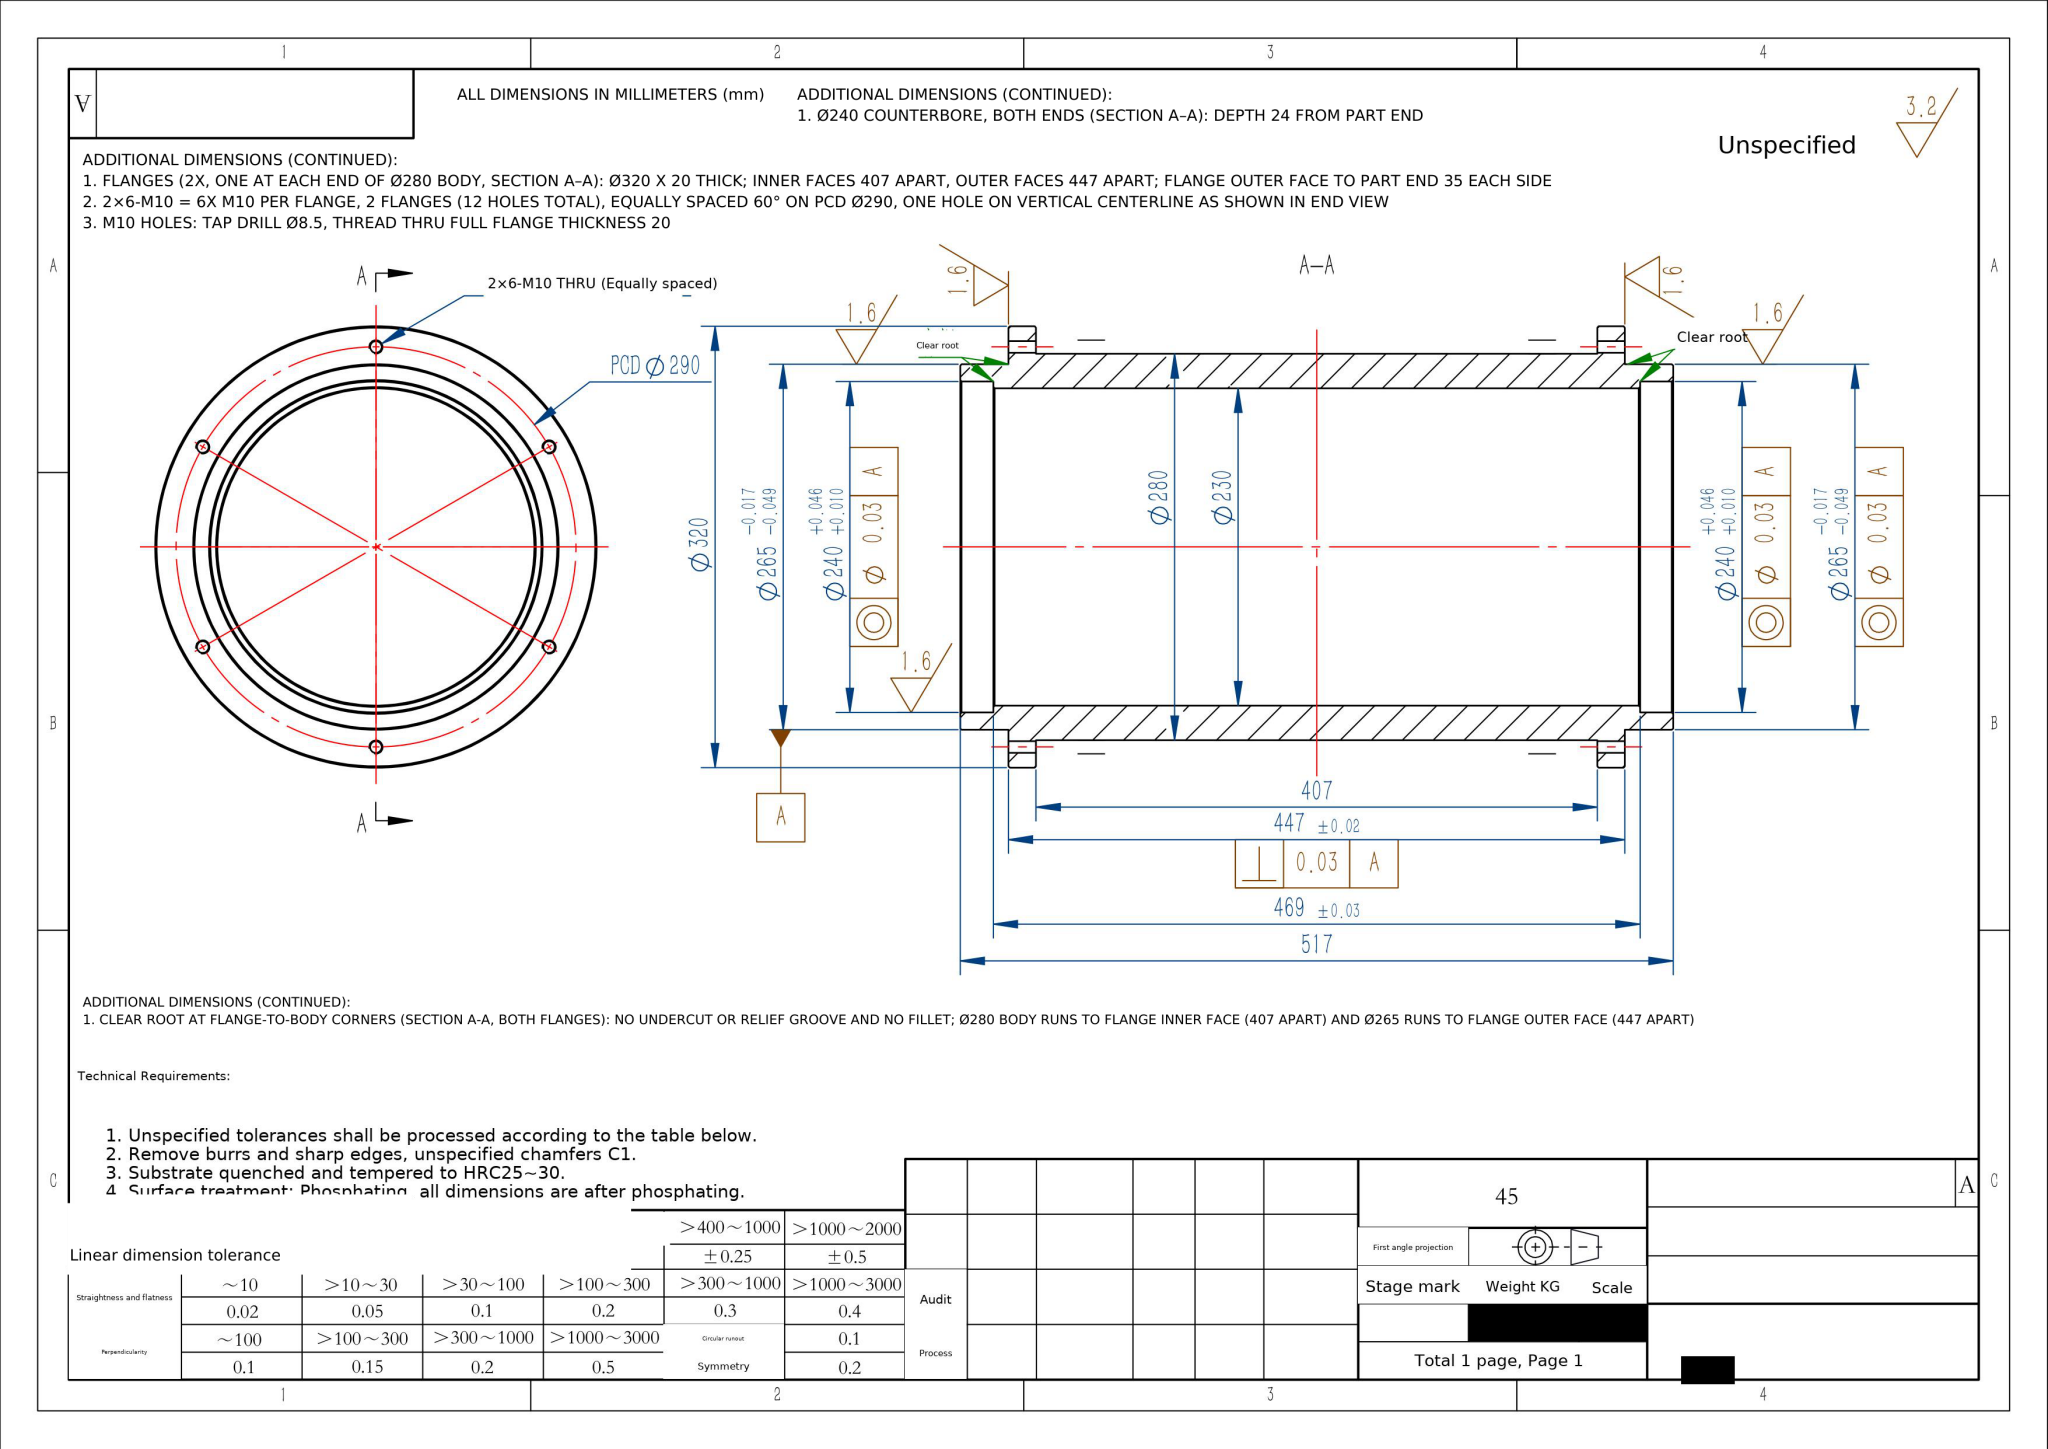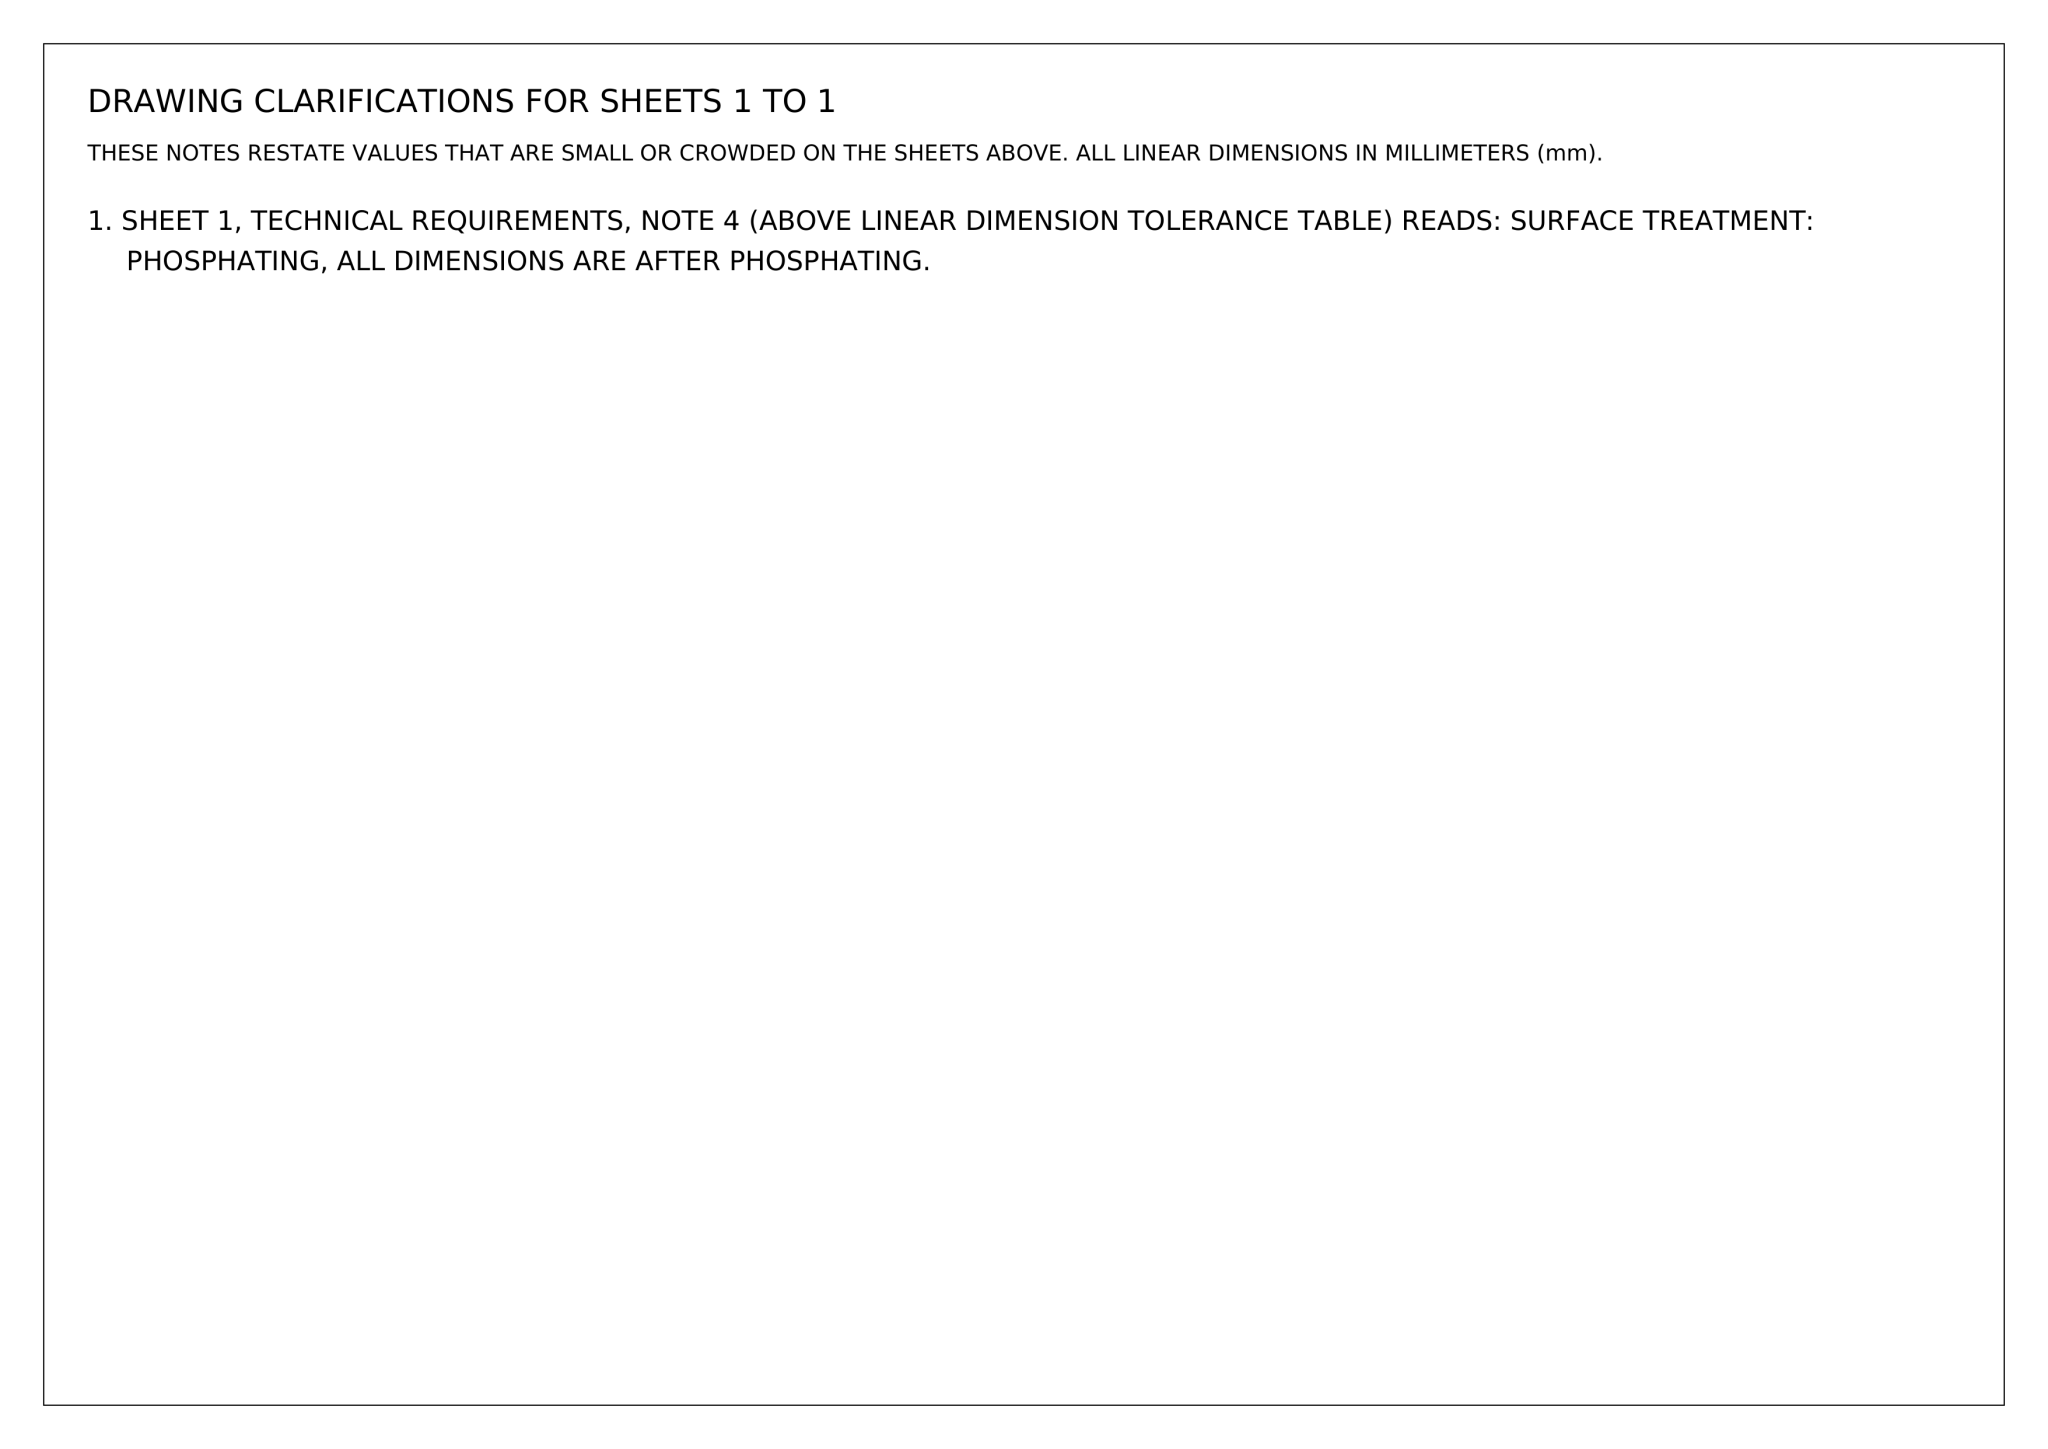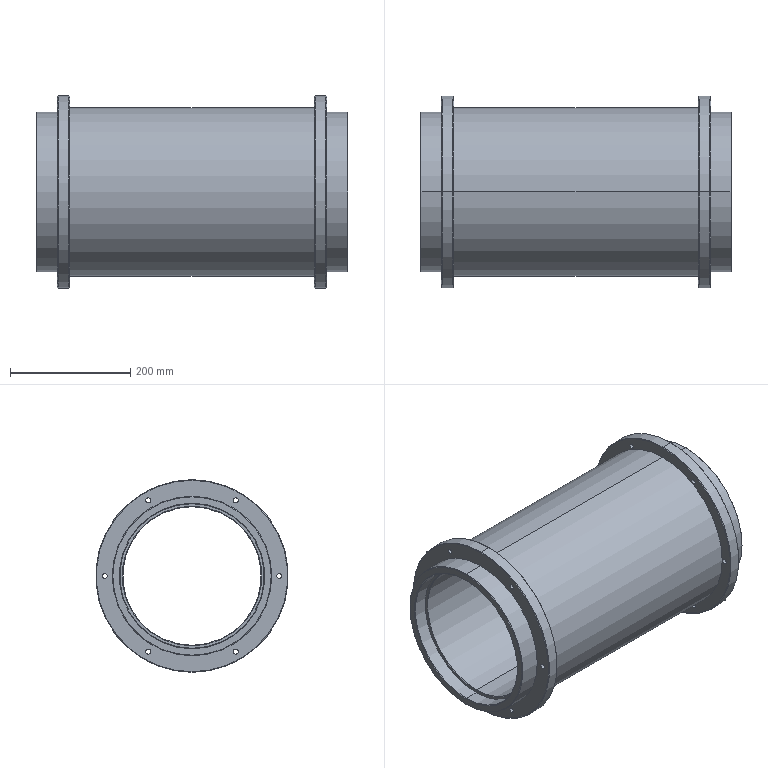Part | NX | mm | 1 solid | 68 faces | box 517 x 320 x 320 mm | volume 10463713 mm3 | cylinder 40 | cone 20 | plane 8 | commonest cylinder face diameters 8.5 x24 240 x4 265 x4 320 x4 230 x2 280 x2